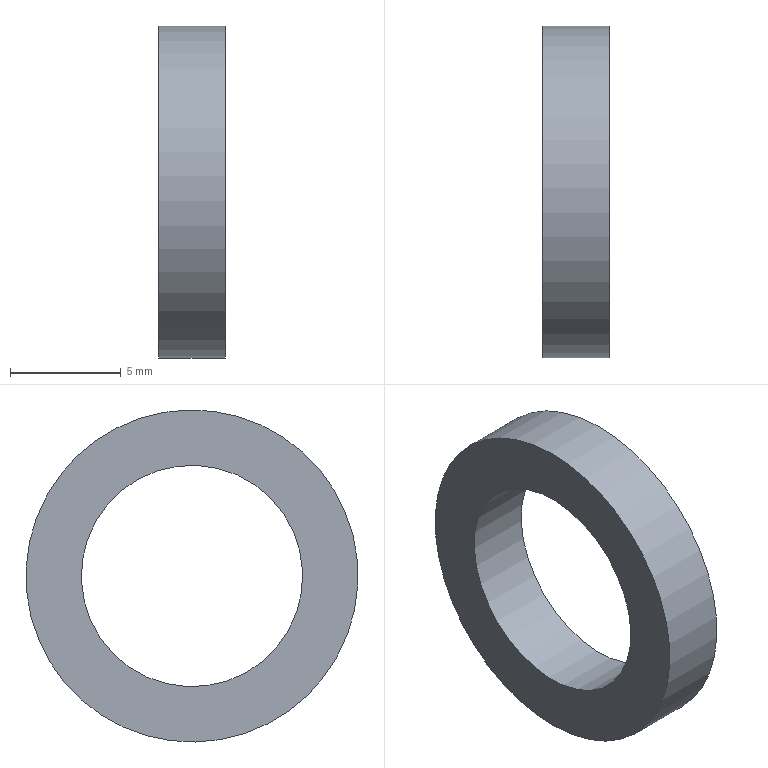Component | NX | 16C__27 | 1 solid | 4 faces | box 3 x 15 x 15 mm | volume 295 mm3 | cylinder 2 | plane 2 | commonest cylinder face diameters 15 x1 10 x1
STEP:
#1=CARTESIAN_POINT('',(0.,0.,0.));
#2=DIRECTION('',(0.,0.,1.));
#3=DIRECTION('',(1.,0.,0.));
#4=AXIS2_PLACEMENT_3D('',#1,#2,#3);
#5=CARTESIAN_POINT('',(65.022,111.966,80.551));
#6=VERTEX_POINT('',#5);
#7=CARTESIAN_POINT('',(65.022,109.608,73.432));
#8=DIRECTION('',(-1.,0.,0.));
#9=DIRECTION('',(0.,0.3144,0.9493));
#10=AXIS2_PLACEMENT_3D('',#7,#8,#9);
#11=CIRCLE('',#10,7.5);
#12=CARTESIAN_POINT('',(65.022,109.608,73.432));
#13=DIRECTION('',(1.,0.,0.));
#14=DIRECTION('',(0.,-0.3144,-0.9493));
#15=AXIS2_PLACEMENT_3D('',#12,#13,#14);
#16=CYLINDRICAL_SURFACE('',#15,7.5);
#17=CARTESIAN_POINT('',(9.425,0.));
#18=DIRECTION('',(-1.,0.));
#19=VECTOR('',#18,1.);
#20=LINE('',#17,#19);
#21=(GEOMETRIC_REPRESENTATION_CONTEXT(2)PARAMETRIC_REPRESENTATION_CONTEXT()REPRESENTATION_CONTEXT('',''));
#22=DEFINITIONAL_REPRESENTATION('',(#20),#21);
#23=PCURVE('',#16,#22);
#24=CARTESIAN_POINT('',(65.022,109.608,73.432));
#25=DIRECTION('',(-1.,0.,0.));
#26=DIRECTION('',(0.,0.3144,0.9493));
#27=AXIS2_PLACEMENT_3D('',#24,#25,#26);
#28=PLANE('',#27);
#29=CARTESIAN_POINT('',(0.,0.));
#30=DIRECTION('',(1.,0.));
#31=AXIS2_PLACEMENT_2D('',#29,#30);
#32=CIRCLE('',#31,7.5);
#33=(GEOMETRIC_REPRESENTATION_CONTEXT(2)PARAMETRIC_REPRESENTATION_CONTEXT()REPRESENTATION_CONTEXT('',''));
#34=DEFINITIONAL_REPRESENTATION('',(#32),#33);
#35=PCURVE('',#28,#34);
#36=SURFACE_CURVE('',#11,(#23,#35),.PCURVE_S1.);
#37=EDGE_CURVE('',#6,#6,#36,.T.);
#38=ORIENTED_EDGE('',*,*,#37,.F.);
#39=CARTESIAN_POINT('',(68.022,111.966,80.551));
#40=VERTEX_POINT('',#39);
#41=CARTESIAN_POINT('',(65.022,111.966,80.551));
#42=CARTESIAN_POINT('',(68.022,111.966,80.551));
#43=B_SPLINE_CURVE_WITH_KNOTS('',1,(#41,#42),.UNSPECIFIED.,.F.,.F.,(2,2),(0.,3.),.PIECEWISE_BEZIER_KNOTS.);
#44=CARTESIAN_POINT('',(9.425,0.));
#45=DIRECTION('',(0.,1.));
#46=VECTOR('',#45,1.);
#47=LINE('',#44,#46);
#48=(GEOMETRIC_REPRESENTATION_CONTEXT(2)PARAMETRIC_REPRESENTATION_CONTEXT()REPRESENTATION_CONTEXT('',''));
#49=DEFINITIONAL_REPRESENTATION('',(#47),#48);
#50=PCURVE('',#16,#49);
#51=CARTESIAN_POINT('',(3.142,0.));
#52=DIRECTION('',(0.,1.));
#53=VECTOR('',#52,1.);
#54=LINE('',#51,#53);
#55=(GEOMETRIC_REPRESENTATION_CONTEXT(2)PARAMETRIC_REPRESENTATION_CONTEXT()REPRESENTATION_CONTEXT('',''));
#56=DEFINITIONAL_REPRESENTATION('',(#54),#55);
#57=PCURVE('',#16,#56);
#58=SEAM_CURVE('',#43,(#50,#57),.PCURVE_S1.);
#59=EDGE_CURVE('',#6,#40,#58,.T.);
#60=ORIENTED_EDGE('',*,*,#59,.T.);
#61=CARTESIAN_POINT('',(68.022,109.608,73.432));
#62=DIRECTION('',(-1.,0.,0.));
#63=DIRECTION('',(0.,0.3144,0.9493));
#64=AXIS2_PLACEMENT_3D('',#61,#62,#63);
#65=CIRCLE('',#64,7.5);
#66=CARTESIAN_POINT('',(9.425,3.));
#67=DIRECTION('',(-1.,0.));
#68=VECTOR('',#67,1.);
#69=LINE('',#66,#68);
#70=(GEOMETRIC_REPRESENTATION_CONTEXT(2)PARAMETRIC_REPRESENTATION_CONTEXT()REPRESENTATION_CONTEXT('',''));
#71=DEFINITIONAL_REPRESENTATION('',(#69),#70);
#72=PCURVE('',#16,#71);
#73=CARTESIAN_POINT('',(68.022,109.608,73.432));
#74=DIRECTION('',(-1.,0.,0.));
#75=DIRECTION('',(0.,0.3144,0.9493));
#76=AXIS2_PLACEMENT_3D('',#73,#74,#75);
#77=PLANE('',#76);
#78=CARTESIAN_POINT('',(0.,0.));
#79=DIRECTION('',(1.,0.));
#80=AXIS2_PLACEMENT_2D('',#78,#79);
#81=CIRCLE('',#80,7.5);
#82=(GEOMETRIC_REPRESENTATION_CONTEXT(2)PARAMETRIC_REPRESENTATION_CONTEXT()REPRESENTATION_CONTEXT('',''));
#83=DEFINITIONAL_REPRESENTATION('',(#81),#82);
#84=PCURVE('',#77,#83);
#85=SURFACE_CURVE('',#65,(#72,#84),.PCURVE_S1.);
#86=EDGE_CURVE('',#40,#40,#85,.T.);
#87=ORIENTED_EDGE('',*,*,#86,.T.);
#88=ORIENTED_EDGE('',*,*,#59,.F.);
#89=EDGE_LOOP('',(#38,#60,#87,#88));
#90=FACE_BOUND('',#89,.T.);
#91=ADVANCED_FACE('',(#90),#16,.T.);
#92=CARTESIAN_POINT('',(65.022,111.18,78.178));
#93=VERTEX_POINT('',#92);
#94=CARTESIAN_POINT('',(65.022,109.608,73.432));
#95=DIRECTION('',(-1.,0.,0.));
#96=DIRECTION('',(0.,0.3144,0.9493));
#97=AXIS2_PLACEMENT_3D('',#94,#95,#96);
#98=CIRCLE('',#97,5.);
#99=CARTESIAN_POINT('',(65.022,109.608,73.432));
#100=DIRECTION('',(1.,0.,0.));
#101=DIRECTION('',(0.,-0.3144,-0.9493));
#102=AXIS2_PLACEMENT_3D('',#99,#100,#101);
#103=CYLINDRICAL_SURFACE('',#102,5.);
#104=CARTESIAN_POINT('',(9.425,0.));
#105=DIRECTION('',(-1.,0.));
#106=VECTOR('',#105,1.);
#107=LINE('',#104,#106);
#108=(GEOMETRIC_REPRESENTATION_CONTEXT(2)PARAMETRIC_REPRESENTATION_CONTEXT()REPRESENTATION_CONTEXT('',''));
#109=DEFINITIONAL_REPRESENTATION('',(#107),#108);
#110=PCURVE('',#103,#109);
#111=CARTESIAN_POINT('',(0.,0.));
#112=DIRECTION('',(1.,-0.));
#113=AXIS2_PLACEMENT_2D('',#111,#112);
#114=CIRCLE('',#113,5.);
#115=(GEOMETRIC_REPRESENTATION_CONTEXT(2)PARAMETRIC_REPRESENTATION_CONTEXT()REPRESENTATION_CONTEXT('',''));
#116=DEFINITIONAL_REPRESENTATION('',(#114),#115);
#117=PCURVE('',#28,#116);
#118=SURFACE_CURVE('',#98,(#110,#117),.PCURVE_S1.);
#119=EDGE_CURVE('',#93,#93,#118,.T.);
#120=ORIENTED_EDGE('',*,*,#119,.F.);
#121=CARTESIAN_POINT('',(68.022,111.18,78.178));
#122=VERTEX_POINT('',#121);
#123=CARTESIAN_POINT('',(65.022,111.18,78.178));
#124=CARTESIAN_POINT('',(68.022,111.18,78.178));
#125=B_SPLINE_CURVE_WITH_KNOTS('',1,(#123,#124),.UNSPECIFIED.,.F.,.F.,(2,2),(0.,3.),.PIECEWISE_BEZIER_KNOTS.);
#126=CARTESIAN_POINT('',(9.425,0.));
#127=DIRECTION('',(0.,1.));
#128=VECTOR('',#127,1.);
#129=LINE('',#126,#128);
#130=(GEOMETRIC_REPRESENTATION_CONTEXT(2)PARAMETRIC_REPRESENTATION_CONTEXT()REPRESENTATION_CONTEXT('',''));
#131=DEFINITIONAL_REPRESENTATION('',(#129),#130);
#132=PCURVE('',#103,#131);
#133=CARTESIAN_POINT('',(3.142,0.));
#134=DIRECTION('',(0.,1.));
#135=VECTOR('',#134,1.);
#136=LINE('',#133,#135);
#137=(GEOMETRIC_REPRESENTATION_CONTEXT(2)PARAMETRIC_REPRESENTATION_CONTEXT()REPRESENTATION_CONTEXT('',''));
#138=DEFINITIONAL_REPRESENTATION('',(#136),#137);
#139=PCURVE('',#103,#138);
#140=SEAM_CURVE('',#125,(#132,#139),.PCURVE_S1.);
#141=EDGE_CURVE('',#93,#122,#140,.T.);
#142=ORIENTED_EDGE('',*,*,#141,.T.);
#143=CARTESIAN_POINT('',(68.022,109.608,73.432));
#144=DIRECTION('',(-1.,0.,0.));
#145=DIRECTION('',(0.,0.3144,0.9493));
#146=AXIS2_PLACEMENT_3D('',#143,#144,#145);
#147=CIRCLE('',#146,5.);
#148=CARTESIAN_POINT('',(9.425,3.));
#149=DIRECTION('',(-1.,0.));
#150=VECTOR('',#149,1.);
#151=LINE('',#148,#150);
#152=(GEOMETRIC_REPRESENTATION_CONTEXT(2)PARAMETRIC_REPRESENTATION_CONTEXT()REPRESENTATION_CONTEXT('',''));
#153=DEFINITIONAL_REPRESENTATION('',(#151),#152);
#154=PCURVE('',#103,#153);
#155=CARTESIAN_POINT('',(0.,0.));
#156=DIRECTION('',(1.,-0.));
#157=AXIS2_PLACEMENT_2D('',#155,#156);
#158=CIRCLE('',#157,5.);
#159=(GEOMETRIC_REPRESENTATION_CONTEXT(2)PARAMETRIC_REPRESENTATION_CONTEXT()REPRESENTATION_CONTEXT('',''));
#160=DEFINITIONAL_REPRESENTATION('',(#158),#159);
#161=PCURVE('',#77,#160);
#162=SURFACE_CURVE('',#147,(#154,#161),.PCURVE_S1.);
#163=EDGE_CURVE('',#122,#122,#162,.T.);
#164=ORIENTED_EDGE('',*,*,#163,.T.);
#165=ORIENTED_EDGE('',*,*,#141,.F.);
#166=EDGE_LOOP('',(#120,#142,#164,#165));
#167=FACE_BOUND('',#166,.F.);
#168=ADVANCED_FACE('',(#167),#103,.F.);
#169=ORIENTED_EDGE('',*,*,#37,.T.);
#170=EDGE_LOOP('',(#169));
#171=FACE_BOUND('',#170,.T.);
#172=ORIENTED_EDGE('',*,*,#119,.F.);
#173=EDGE_LOOP('',(#172));
#174=FACE_BOUND('',#173,.T.);
#175=ADVANCED_FACE('',(#171,#174),#28,.T.);
#176=ORIENTED_EDGE('',*,*,#86,.F.);
#177=EDGE_LOOP('',(#176));
#178=FACE_BOUND('',#177,.T.);
#179=ORIENTED_EDGE('',*,*,#163,.T.);
#180=EDGE_LOOP('',(#179));
#181=FACE_BOUND('',#180,.T.);
#182=ADVANCED_FACE('',(#178,#181),#77,.F.);
#183=CLOSED_SHELL('',(#91,#168,#175,#182));
#184=MANIFOLD_SOLID_BREP('',#183);
#185=(LENGTH_UNIT()NAMED_UNIT(*)SI_UNIT(.MILLI.,.METRE.));
#186=UNCERTAINTY_MEASURE_WITH_UNIT(LENGTH_MEASURE(0.00001),#185,'','');
#187=(NAMED_UNIT(*)PLANE_ANGLE_UNIT()SI_UNIT($,.RADIAN.));
#188=(NAMED_UNIT(*)SI_UNIT($,.STERADIAN.)SOLID_ANGLE_UNIT());
#189=(GEOMETRIC_REPRESENTATION_CONTEXT(3)GLOBAL_UNCERTAINTY_ASSIGNED_CONTEXT((#186))GLOBAL_UNIT_ASSIGNED_CONTEXT((#185,#187,#188))REPRESENTATION_CONTEXT('',''));
#190=ADVANCED_BREP_SHAPE_REPRESENTATION('',(#4,#184),#189);